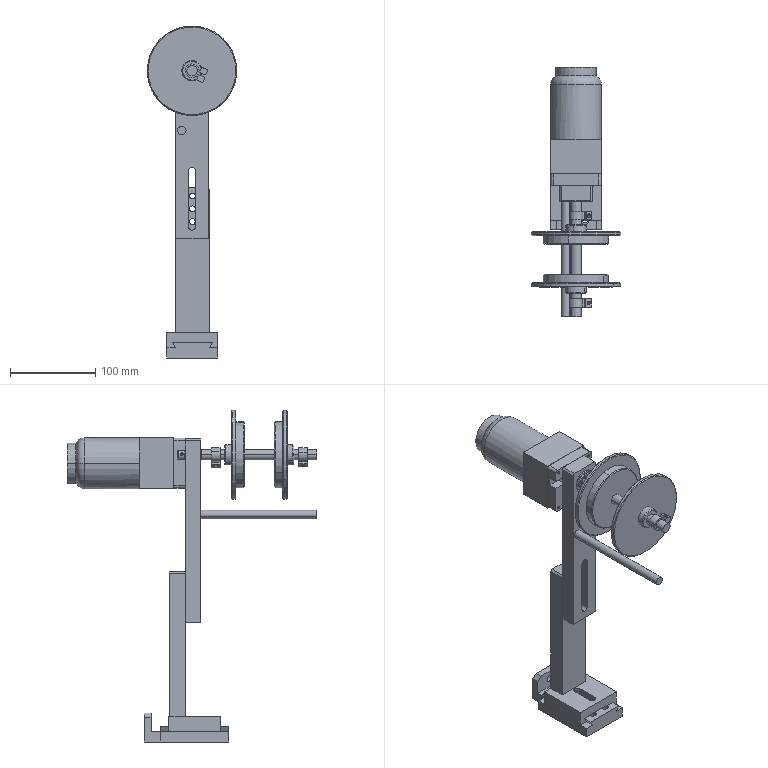Assembly | SolidWorks | mm | 15 component files | 15 solids | 503 faces | box 105 x 293 x 389.5 mm | volume 999952 mm3 | cylinder 187 | plane 136 | torus 102 | sphere 52 | cone 26 | commonest cylinder face diameters 12 x14 4.5 x12 6.8 x10 11 x10 6.5 x10 8 x10 4.2 x8 9 x8
Bill of materials:
AdjustmentBlock | 1 |  | L-shaped (stepped) prismatic block: a tall upright plate with two chamfered upper corners and a lower, forward-projecting step. The upright carries one larger through hole; the step carries two smaller through holes parallel to it.
Axis1 | 1 |  | Plain solid round rod/pin with flat ends and a constant diameter along its length.
deep groove ball bearings gb | 2 |  | Annular assembly that looks like a radial ball bearing: an outer ring, an inner ring with a central bore, and a single row of about 12 spheres between them.
DovetailBase1 | 1 |  | Rectangular plate with a raised dovetail-profile tongue running its full length on top. It has five through holes: four smaller holes in a rectangular pattern and one larger central hole.
DovetailBase2 | 1 |  | Square block with a dovetail-profile groove running through its underside. The top face has one long straight slot with rounded ends and two round through holes.
FixedBlock | 1 |  | Long rectangular bar with three small round through holes in a line near one end. Its top end edges have small chamfers.
FixedBlock2 | 1 |  | Long flat bar with features along its length: a large round hole near one end, two small holes below it, one medium off-centre hole, and a long slot with rounded ends near the other end.
Motor2IK6GN-C | 1 |  | Unit that looks like a geared motor: a square box-shaped front housing with four corner holes on its face, a protruding round output shaft with a short boss, and a cylindrical body behind with a rounded rear edge and a smaller rear end cap.
MotorAxis | 1 |  | Solid round rod/shaft with two narrow circumferential grooves near one end. Otherwise it has a constant diameter.
MotorPlate | 1 | 6061 Alloy | Thick square plate with rounded corners. It has a large round bore placed off-centre toward one edge, four small corner holes and two medium holes below the bore. The isometric view also shows a slot cut from one side edge into the bore.
RubberStopWheel | 2 |  | Turned stepped disc, all on one axis: a thin large-diameter flange, a wider and thicker raised boss on one face, a small short hub on the opposite face, and a small central through hole.
TAR-02-038ShaftClampBlock | 2 |  | Split-ring clamp shape: a thick round ring split on one side. The split continues between two parallel rectangular tabs, which are separated by a gap. One straight round hole passes through both tabs across the gap. There are rounded relief notches where the tabs meet the ring.
Mates:
1. coincident | DovetailBase1-1 face at (-48.047, -14.04, 9) dir (0, 0, 1) | DovetailBase2-1 face at (-24.583, -56.04, 9) dir (0, 0, -1)
2. coincident | DovetailBase1-1 face at (-38.243, -58.04, -14.66) dir (0.866, 0, -0.5) | DovetailBase2-1 face at (-28.047, -56.04, 3) dir (-0.866, 0, 0.5)
3. coincident | DovetailBase1-1 face at (-78.047, 25.96, 9) dir (0, 1, 0) | AdjustmentBlock-1 face at (-48.047, 25.96, 8) dir (0, -1, 0)
4. concentric | DovetailBase1-1 edge at (-58.047, 25.96, -2) dir (0, 1, 0) r 2.1 | AdjustmentBlock-1 face at (-58.047, 44.96, -2) dir (0, 1, 0) r 3.25
5. concentric | DovetailBase1-1 face at (-38.047, 25.96, -2) dir (0, 1, 0) r 2.1 | AdjustmentBlock-1 face at (-38.047, 44.96, -2) dir (0, 1, 0) r 3.25
6. coincident | DovetailBase2-1 face at (-48.047, -14.04, 21) dir (0, 0, 1) | FixedBlock-1 face at (-67.547, -3.54, 21) dir (0, 0, -1)
7. concentric | DovetailBase2-1 face at (-38.047, 5.96, 9.3) dir (0, 0, -1) r 3.25 | FixedBlock-1 face at (-38.047, 5.96, 21) dir (0, 0, -1) r 2.5
8. concentric | DovetailBase2-1 face at (-58.047, 5.96, 9.3) dir (0, 0, -1) r 3.25 | FixedBlock-1 face at (-58.047, 5.96, 21) dir (0, 0, -1) r 2.5
9. concentric | FixedBlock2-1 face at (-48.547, -11.54, 328) dir (0, 1, 0) r 14 | MotorPlate-1 face at (-48.547, 10.46, 328) dir (0, -1, 0) r 16
10. coincident | FixedBlock2-1 face at (-48.547, -3.54, 239) dir (0, 1, 0) | MotorPlate-1 face at (-19.047, -3.54, 288.5) dir (0, -1, 0)
11. parallel | FixedBlock2-1 face at (-67.547, -3.54, 131) dir (-1, 0, 0) | MotorPlate-1 face at (-78.047, 10.46, 347.5) dir (-1, 0, 0)
12. coincident | MotorPlate-1 face at (-19.047, 10.46, 288.5) dir (0, 1, 0) | Motor2IK6GN-C-1 face at (-18.547, 10.46, 288) dir (0, -1, 0)
13. concentric | MotorPlate-1 face at (-48.547, 10.46, 328) dir (0, -1, 0) r 16 | Motor2IK6GN-C-1 face at (-48.547, 7.46, 328) dir (0, 1, 0) r 12
14. parallel | MotorPlate-1 face at (-78.047, 10.46, 347.5) dir (-1, 0, 0) | Motor2IK6GN-C-1 face at (-78.547, 50.46, 348) dir (-1, 0, 0)
15. coincident | FixedBlock-1 face at (-48.047, -3.54, 106) dir (0, -1, 0) | FixedBlock2-1 face at (-48.547, -3.54, 239) dir (0, 1, 0)
16. coincident | FixedBlock-1 face at (-67.547, -3.54, 21) dir (-1, 0, 0) | FixedBlock2-1 face at (-67.547, -3.54, 131) dir (-1, 0, 0)
17. concentric | FixedBlock2-1 face at (-48.547, -13.54, 328) dir (0, -1, 0) r 14 | MotorAxis-1 face at (-48.547, -157.54, 328) dir (0, 1, 0) r 6
18. concentric | FixedBlock2-1 face at (-48.547, -13.54, 328) dir (0, -1, 0) r 14 | deep groove ball bearings gb-1 face at (-48.547, -8.829, 328) dir (0, 1, 0) r 13
19. coincident | FixedBlock2-1 face at (-48.547, -21.54, 239) dir (0, -1, 0) | deep groove ball bearings gb-1 edge at (-48.547, -21.54, 328) dir (0, -1, 0) r 12.5
20. concentric | FixedBlock2-1 face at (-48.547, -11.54, 328) dir (0, 1, 0) r 14 | deep groove ball bearings gb-2 face at (-48.547, -16.25, 328) dir (0, -1, 0) r 13
21. coincident | FixedBlock2-1 face at (-48.547, -11.54, 328) dir (0, 1, 0) | deep groove ball bearings gb-2 face at (-61.547, -11.54, 328) dir (0, -1, 0)
22. coincident | FixedBlock2-1 face at (-48.547, -21.54, 239) dir (0, -1, 0) | MotorAxis-1 face at (-43.168, -21.54, 327.529) dir (0, -1, 0)
23. concentric | MotorAxis-1 face at (-48.547, -157.54, 328) dir (0, 1, 0) r 6 | RubberStopWheel-1 face at (-48.547, 26.502, 328) dir (0, -1, 0) r 6
24. concentric | MotorAxis-1 face at (-48.547, -157.54, 328) dir (0, 1, 0) r 6 | RubberStopWheel-2 face at (-48.547, -206.498, 328) dir (0, 1, 0) r 6
25. distance | RubberStopWheel-1 face at (-48.547, -62.498, 328) dir (0, -1, 0) | RubberStopWheel-2 face at (-48.547, -117.498, 328) dir (0, 1, 0)
26. distance | DovetailBase1-1 face at (-78.047, -54.04, 9) dir (0, -1, 0) | DovetailBase2-1 face at (-18.047, -44.04, 3) dir (0, -1, 0)
27. concentric | MotorAxis-1 face at (-48.547, -157.54, 328) dir (0, 1, 0) r 6 | TAR-02-038ShaftClampBlock-2 face at (-48.547, -33.909, 328) dir (0, -1, 0) r 6
28. concentric | MotorAxis-1 face at (-48.547, -157.54, 328) dir (0, 1, 0) r 6 | TAR-02-038ShaftClampBlock-1 face at (-48.547, -136.199, 328) dir (0, -1, 0) r 6
29. distance | FixedBlock2-1 face at (-67.547, -3.54, 131) dir (0, 0, -1) | FixedBlock-1 face at (-67.547, -3.54, 191) dir (0, 0, 1)
30. concentric | FixedBlock2-1 face at (-60.547, -3.54, 258) dir (0, 1, 0) r 3.25 | Axis1-1 face at (-60.547, -157.54, 258) dir (0, 1, 0) r 5
31. coincident | FixedBlock2-1 face at (-48.547, -21.54, 239) dir (0, -1, 0) | Axis1-1 face at (-60.547, -21.54, 258) dir (0, 1, 0)